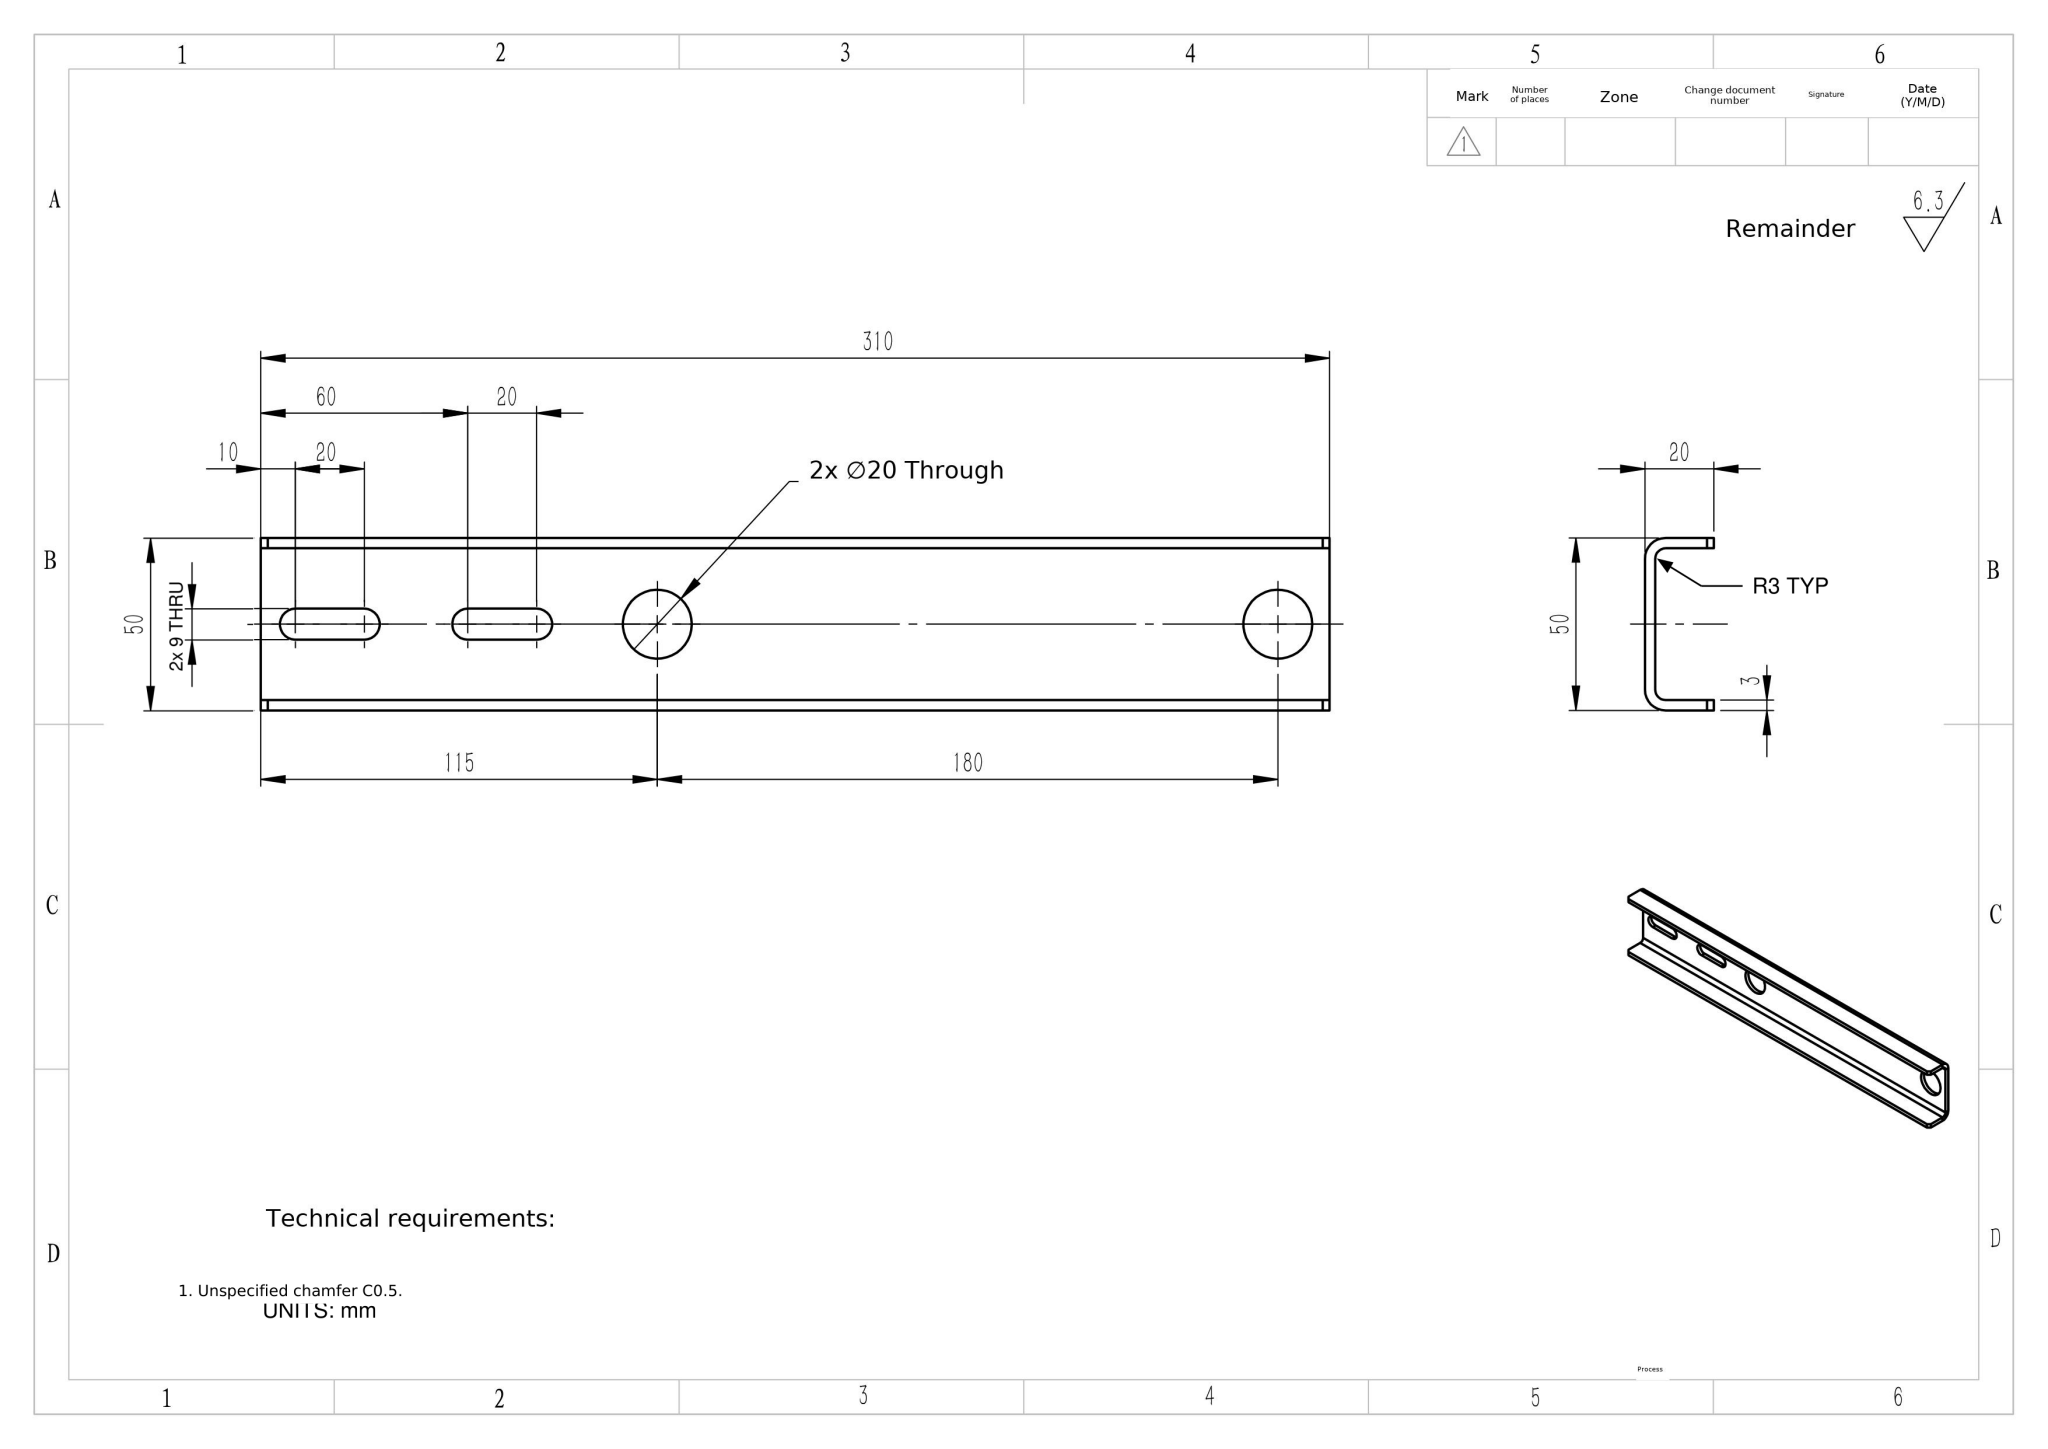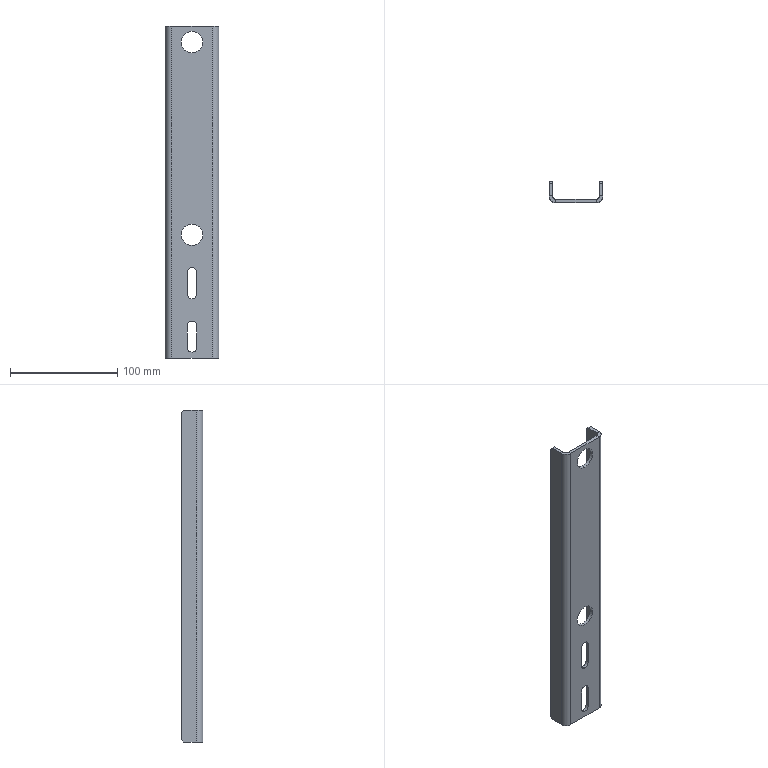Part | NX | mm | 1 solid | 40 faces | box 50 x 20 x 310 mm | volume 71157 mm3 | plane 26 | cylinder 14 | commonest cylinder face diameters 9 x6 20 x4 12 x2 6 x2